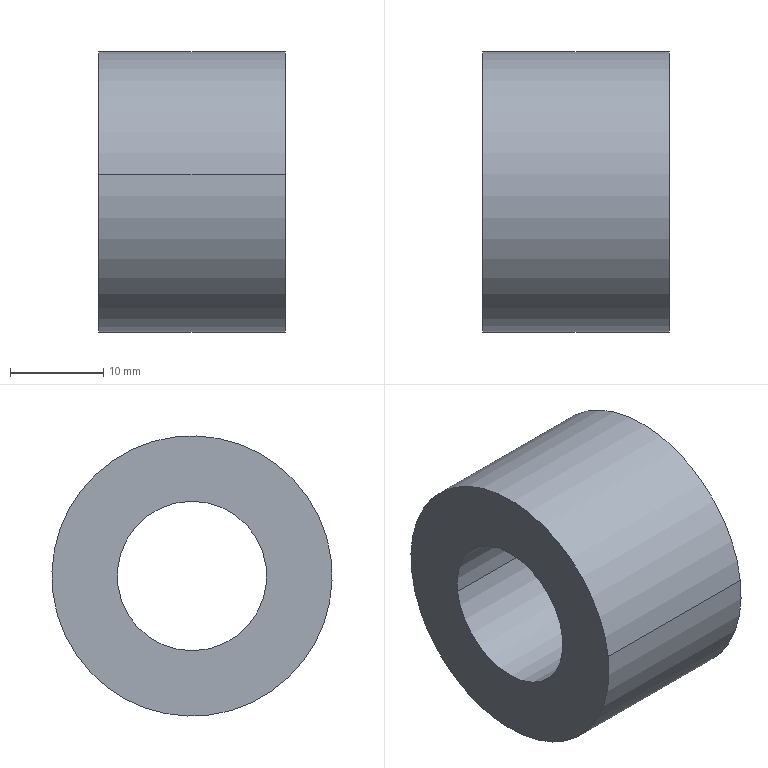Component | SolidWorks | MotorPulley1-1 | 1 solid | 6 faces | box 20 x 30 x 30 mm | volume 10116 mm3 | cylinder 4 | plane 2 | commonest cylinder face diameters 16 x2 30 x2
build123d program:
from build123d import *

# Parameters (mm, degrees)
SKETCH1_R           = 15
SKETCH1_R_2         = 8
BOSS_EXTRUDE1_DEPTH = 20


with BuildPart() as part:
    # Sketch1 → Boss-Extrude1 (new body)
    with BuildSketch(Plane.XY):
        Circle(SKETCH1_R)
        Circle(SKETCH1_R_2, mode=Mode.SUBTRACT)
    extrude(amount=BOSS_EXTRUDE1_DEPTH)


solid = part.part

# Placed as in the assembly
solid = solid.moved(Location((-254.371, -367.407, 334), (0, 90, 0)))
STEP:
#1=CARTESIAN_POINT('',(-9.227,-14.152,13.11));
#2=VERTEX_POINT('',#1);
#3=CARTESIAN_POINT('',(-9.227,-14.777,13.189));
#4=VERTEX_POINT('',#3);
#5=CARTESIAN_POINT('',(-9.227,-14.465,13.15));
#6=DIRECTION('',(1.,-0.,-0.));
#7=DIRECTION('',(0.,-0.992,0.126));
#8=AXIS2_PLACEMENT_3D('',#5,#6,#7);
#9=CIRCLE('',#8,0.315);
#10=EDGE_CURVE('',#2,#4,#9,.T.);
#11=ORIENTED_EDGE('',*,*,#10,.T.);
#12=CARTESIAN_POINT('',(-10.015,-14.777,13.189));
#13=VERTEX_POINT('',#12);
#14=CARTESIAN_POINT('',(-9.227,-14.777,13.189));
#15=DIRECTION('',(-1.,0.,0.));
#16=VECTOR('',#15,39.37);
#17=LINE('',#14,#16);
#18=EDGE_CURVE('',#4,#13,#17,.T.);
#19=ORIENTED_EDGE('',*,*,#18,.T.);
#20=CARTESIAN_POINT('',(-10.015,-14.152,13.11));
#21=VERTEX_POINT('',#20);
#22=CARTESIAN_POINT('',(-10.015,-14.465,13.15));
#23=DIRECTION('',(1.,-0.,-0.));
#24=DIRECTION('',(0.,-0.992,0.126));
#25=AXIS2_PLACEMENT_3D('',#22,#23,#24);
#26=CIRCLE('',#25,0.315);
#27=EDGE_CURVE('',#21,#13,#26,.T.);
#28=ORIENTED_EDGE('',*,*,#27,.F.);
#29=CARTESIAN_POINT('',(-9.227,-14.152,13.11));
#30=DIRECTION('',(-1.,0.,0.));
#31=VECTOR('',#30,39.37);
#32=LINE('',#29,#31);
#33=EDGE_CURVE('',#2,#21,#32,.T.);
#34=ORIENTED_EDGE('',*,*,#33,.F.);
#35=EDGE_LOOP('',(#11,#19,#28,#34));
#36=FACE_OUTER_BOUND('',#35,.T.);
#37=CARTESIAN_POINT('',(-9.227,-14.465,13.15));
#38=DIRECTION('',(-1.,0.,0.));
#39=DIRECTION('',(0.,0.992,-0.126));
#40=AXIS2_PLACEMENT_3D('',#37,#38,#39);
#41=CYLINDRICAL_SURFACE('',#40,0.315);
#42=ADVANCED_FACE('',(#36),#41,.F.);
#43=CARTESIAN_POINT('',(-9.227,-15.051,13.224));
#44=VERTEX_POINT('',#43);
#45=CARTESIAN_POINT('',(-9.227,-13.879,13.075));
#46=VERTEX_POINT('',#45);
#47=CARTESIAN_POINT('',(-9.227,-14.465,13.15));
#48=DIRECTION('',(1.,-0.,-0.));
#49=DIRECTION('',(0.,-0.992,0.126));
#50=AXIS2_PLACEMENT_3D('',#47,#48,#49);
#51=CIRCLE('',#50,0.5906);
#52=EDGE_CURVE('',#44,#46,#51,.T.);
#53=ORIENTED_EDGE('',*,*,#52,.F.);
#54=CARTESIAN_POINT('',(-10.015,-15.051,13.224));
#55=VERTEX_POINT('',#54);
#56=CARTESIAN_POINT('',(-9.227,-15.051,13.224));
#57=DIRECTION('',(-1.,0.,0.));
#58=VECTOR('',#57,39.37);
#59=LINE('',#56,#58);
#60=EDGE_CURVE('',#44,#55,#59,.T.);
#61=ORIENTED_EDGE('',*,*,#60,.T.);
#62=CARTESIAN_POINT('',(-10.015,-13.879,13.075));
#63=VERTEX_POINT('',#62);
#64=CARTESIAN_POINT('',(-10.015,-14.465,13.15));
#65=DIRECTION('',(1.,-0.,-0.));
#66=DIRECTION('',(0.,-0.992,0.126));
#67=AXIS2_PLACEMENT_3D('',#64,#65,#66);
#68=CIRCLE('',#67,0.5906);
#69=EDGE_CURVE('',#55,#63,#68,.T.);
#70=ORIENTED_EDGE('',*,*,#69,.T.);
#71=CARTESIAN_POINT('',(-9.227,-13.879,13.075));
#72=DIRECTION('',(-1.,0.,0.));
#73=VECTOR('',#72,39.37);
#74=LINE('',#71,#73);
#75=EDGE_CURVE('',#46,#63,#74,.T.);
#76=ORIENTED_EDGE('',*,*,#75,.F.);
#77=EDGE_LOOP('',(#53,#61,#70,#76));
#78=FACE_OUTER_BOUND('',#77,.T.);
#79=CARTESIAN_POINT('',(-9.227,-14.465,13.15));
#80=DIRECTION('',(-1.,0.,0.));
#81=DIRECTION('',(0.,0.992,-0.126));
#82=AXIS2_PLACEMENT_3D('',#79,#80,#81);
#83=CYLINDRICAL_SURFACE('',#82,0.5906);
#84=ADVANCED_FACE('',(#78),#83,.T.);
#85=CARTESIAN_POINT('',(-9.227,-14.465,13.15));
#86=DIRECTION('',(1.,-0.,-0.));
#87=DIRECTION('',(0.,-0.992,0.126));
#88=AXIS2_PLACEMENT_3D('',#85,#86,#87);
#89=CIRCLE('',#88,0.5906);
#90=EDGE_CURVE('',#46,#44,#89,.T.);
#91=ORIENTED_EDGE('',*,*,#90,.T.);
#92=ORIENTED_EDGE('',*,*,#52,.T.);
#93=EDGE_LOOP('',(#91,#92));
#94=FACE_OUTER_BOUND('',#93,.T.);
#95=ORIENTED_EDGE('',*,*,#10,.F.);
#96=CARTESIAN_POINT('',(-9.227,-14.465,13.15));
#97=DIRECTION('',(1.,-0.,-0.));
#98=DIRECTION('',(0.,-0.992,0.126));
#99=AXIS2_PLACEMENT_3D('',#96,#97,#98);
#100=CIRCLE('',#99,0.315);
#101=EDGE_CURVE('',#4,#2,#100,.T.);
#102=ORIENTED_EDGE('',*,*,#101,.F.);
#103=EDGE_LOOP('',(#95,#102));
#104=FACE_BOUND('',#103,.T.);
#105=CARTESIAN_POINT('',(-9.227,-14.465,13.15));
#106=DIRECTION('',(1.,-0.,-0.));
#107=DIRECTION('',(-0.,-0.992,0.126));
#108=AXIS2_PLACEMENT_3D('',#105,#106,#107);
#109=PLANE('',#108);
#110=ADVANCED_FACE('',(#94,#104),#109,.T.);
#111=CARTESIAN_POINT('',(-10.015,-14.465,13.15));
#112=DIRECTION('',(1.,-0.,-0.));
#113=DIRECTION('',(0.,-0.992,0.126));
#114=AXIS2_PLACEMENT_3D('',#111,#112,#113);
#115=CIRCLE('',#114,0.5906);
#116=EDGE_CURVE('',#63,#55,#115,.T.);
#117=ORIENTED_EDGE('',*,*,#116,.F.);
#118=ORIENTED_EDGE('',*,*,#69,.F.);
#119=EDGE_LOOP('',(#117,#118));
#120=FACE_OUTER_BOUND('',#119,.T.);
#121=ORIENTED_EDGE('',*,*,#27,.T.);
#122=CARTESIAN_POINT('',(-10.015,-14.465,13.15));
#123=DIRECTION('',(1.,-0.,-0.));
#124=DIRECTION('',(0.,-0.992,0.126));
#125=AXIS2_PLACEMENT_3D('',#122,#123,#124);
#126=CIRCLE('',#125,0.315);
#127=EDGE_CURVE('',#13,#21,#126,.T.);
#128=ORIENTED_EDGE('',*,*,#127,.T.);
#129=EDGE_LOOP('',(#121,#128));
#130=FACE_BOUND('',#129,.T.);
#131=CARTESIAN_POINT('',(-10.015,-14.465,13.15));
#132=DIRECTION('',(1.,-0.,-0.));
#133=DIRECTION('',(-0.,-0.992,0.126));
#134=AXIS2_PLACEMENT_3D('',#131,#132,#133);
#135=PLANE('',#134);
#136=ADVANCED_FACE('',(#120,#130),#135,.F.);
#137=ORIENTED_EDGE('',*,*,#60,.F.);
#138=ORIENTED_EDGE('',*,*,#90,.F.);
#139=ORIENTED_EDGE('',*,*,#75,.T.);
#140=ORIENTED_EDGE('',*,*,#116,.T.);
#141=EDGE_LOOP('',(#137,#138,#139,#140));
#142=FACE_OUTER_BOUND('',#141,.T.);
#143=CARTESIAN_POINT('',(-9.227,-14.465,13.15));
#144=DIRECTION('',(-1.,0.,0.));
#145=DIRECTION('',(0.,0.992,-0.126));
#146=AXIS2_PLACEMENT_3D('',#143,#144,#145);
#147=CYLINDRICAL_SURFACE('',#146,0.5906);
#148=ADVANCED_FACE('',(#142),#147,.T.);
#149=ORIENTED_EDGE('',*,*,#18,.F.);
#150=ORIENTED_EDGE('',*,*,#101,.T.);
#151=ORIENTED_EDGE('',*,*,#33,.T.);
#152=ORIENTED_EDGE('',*,*,#127,.F.);
#153=EDGE_LOOP('',(#149,#150,#151,#152));
#154=FACE_OUTER_BOUND('',#153,.T.);
#155=CARTESIAN_POINT('',(-9.227,-14.465,13.15));
#156=DIRECTION('',(-1.,0.,0.));
#157=DIRECTION('',(0.,0.992,-0.126));
#158=AXIS2_PLACEMENT_3D('',#155,#156,#157);
#159=CYLINDRICAL_SURFACE('',#158,0.315);
#160=ADVANCED_FACE('',(#154),#159,.F.);
#161=CLOSED_SHELL('',(#42,#84,#110,#136,#148,#160));
#162=MANIFOLD_SOLID_BREP('',#161);
#163=CARTESIAN_POINT('',(0.,0.,0.));
#164=DIRECTION('',(0.,0.,1.));
#165=DIRECTION('',(1.,0.,0.));
#166=AXIS2_PLACEMENT_3D('',#163,#164,#165);
#167=(LENGTH_UNIT()NAMED_UNIT(*)SI_UNIT($,.METRE.));
#168=LENGTH_MEASURE_WITH_UNIT(LENGTH_MEASURE(0.0254),#167);
#169=DIMENSIONAL_EXPONENTS(1.,0.,0.,0.,0.,0.,0.);
#170=(CONVERSION_BASED_UNIT('',#168)LENGTH_UNIT()NAMED_UNIT(#169));
#171=UNCERTAINTY_MEASURE_WITH_UNIT(LENGTH_MEASURE(0.00001),#170,'','');
#172=(NAMED_UNIT(*)PLANE_ANGLE_UNIT()SI_UNIT($,.RADIAN.));
#173=(NAMED_UNIT(*)SI_UNIT($,.STERADIAN.)SOLID_ANGLE_UNIT());
#174=(GEOMETRIC_REPRESENTATION_CONTEXT(3)GLOBAL_UNCERTAINTY_ASSIGNED_CONTEXT((#171))GLOBAL_UNIT_ASSIGNED_CONTEXT((#170,#172,#173))REPRESENTATION_CONTEXT('',''));
#175=ADVANCED_BREP_SHAPE_REPRESENTATION('',(#162,#166),#174);
#176=COLOUR_RGB('',0.7922,0.8196,0.9333);
#177=FILL_AREA_STYLE_COLOUR('',#176);
#178=FILL_AREA_STYLE('',(#177));
#179=SURFACE_STYLE_FILL_AREA(#178);
#180=SURFACE_SIDE_STYLE('',(#179));
#181=SURFACE_STYLE_USAGE(.BOTH.,#180);
#182=PRESENTATION_STYLE_ASSIGNMENT((#181));
#183=STYLED_ITEM('',(#182),#162);
#184=PRESENTATION_LAYER_ASSIGNMENT('','',(#183));
#185=(LENGTH_UNIT()NAMED_UNIT(*)SI_UNIT($,.METRE.));
#186=LENGTH_MEASURE_WITH_UNIT(LENGTH_MEASURE(0.0254),#185);
#187=DIMENSIONAL_EXPONENTS(1.,0.,0.,0.,0.,0.,0.);
#188=(CONVERSION_BASED_UNIT('',#186)LENGTH_UNIT()NAMED_UNIT(#187));
#189=UNCERTAINTY_MEASURE_WITH_UNIT(LENGTH_MEASURE(0.00001),#188,'','');
#190=(NAMED_UNIT(*)PLANE_ANGLE_UNIT()SI_UNIT($,.RADIAN.));
#191=(NAMED_UNIT(*)SI_UNIT($,.STERADIAN.)SOLID_ANGLE_UNIT());
#192=(GEOMETRIC_REPRESENTATION_CONTEXT(3)GLOBAL_UNCERTAINTY_ASSIGNED_CONTEXT((#189))GLOBAL_UNIT_ASSIGNED_CONTEXT((#188,#190,#191))REPRESENTATION_CONTEXT('',''));
#193=MECHANICAL_DESIGN_GEOMETRIC_PRESENTATION_REPRESENTATION('',(#183),#192);